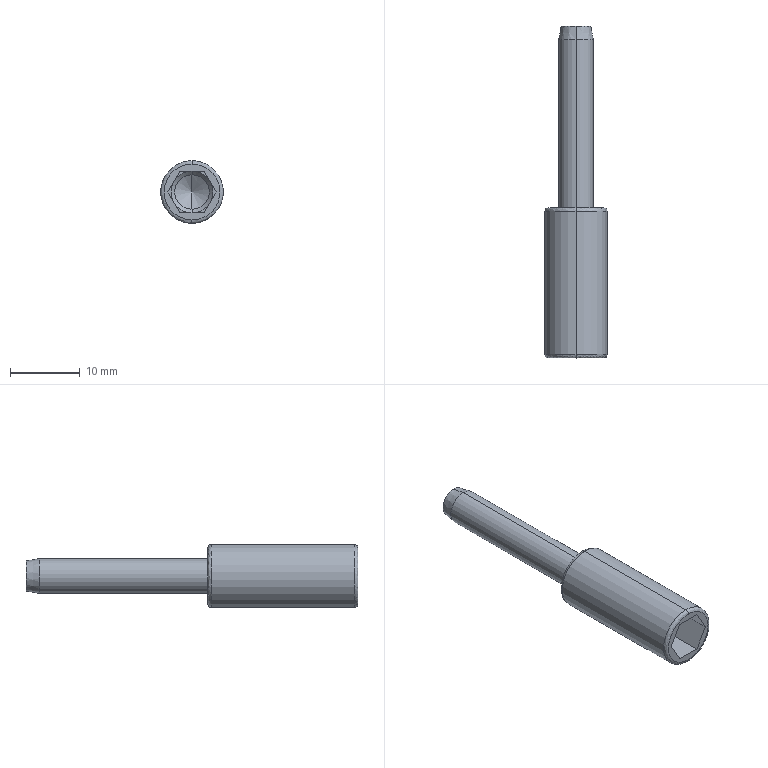Component | SolidWorks | HZ022-SE32x25S-1_HZ022-SE32x25S (10)-1 | 1 solid | 31 faces | box 9 x 47.5 x 9 mm | volume 1481 mm3 | plane 15 | cylinder 6 | cone 6 | spline 4 | commonest cylinder face diameters 9 x2 5 x2 4.917 x2 | material AL6061
STEP:
#1=COLOUR_RGB('',0.7922,0.8196,0.9333);
#2=FILL_AREA_STYLE_COLOUR('',#1);
#3=FILL_AREA_STYLE('',(#2));
#4=SURFACE_STYLE_FILL_AREA(#3);
#5=SURFACE_SIDE_STYLE('',(#4));
#6=SURFACE_STYLE_USAGE(.BOTH.,#5);
#7=PRESENTATION_STYLE_ASSIGNMENT((#6));
#8=CARTESIAN_POINT('',(-1.146,-5.555,13.976));
#9=VERTEX_POINT('',#8);
#10=CARTESIAN_POINT('',(-1.146,-5.555,13.661));
#11=VERTEX_POINT('',#10);
#12=CARTESIAN_POINT('',(-1.146,-5.555,13.976));
#13=CARTESIAN_POINT('',(-0.8313,-5.555,13.976));
#14=CARTESIAN_POINT('',(-0.8313,-5.555,13.661));
#15=CARTESIAN_POINT('',(-1.146,-5.555,13.661));
#16=(BOUNDED_CURVE()B_SPLINE_CURVE(3,(#12,#13,#14,#15),.UNSPECIFIED.,.F.,.F.)B_SPLINE_CURVE_WITH_KNOTS((4,4),(0.,1.),.UNSPECIFIED.)CURVE()GEOMETRIC_REPRESENTATION_ITEM()RATIONAL_B_SPLINE_CURVE((1.,0.3333,0.3333,1.))REPRESENTATION_ITEM(''));
#17=EDGE_CURVE('',#9,#11,#16,.T.);
#18=ORIENTED_EDGE('',*,*,#17,.T.);
#19=CARTESIAN_POINT('',(-1.146,-5.536,13.642));
#20=VERTEX_POINT('',#19);
#21=CARTESIAN_POINT('',(-1.146,-5.536,13.661));
#22=DIRECTION('',(1.,-0.,-0.));
#23=DIRECTION('',(0.,0.,-1.));
#24=AXIS2_PLACEMENT_3D('',#21,#22,#23);
#25=CIRCLE('',#24,0.01969);
#26=EDGE_CURVE('',#11,#20,#25,.T.);
#27=ORIENTED_EDGE('',*,*,#26,.T.);
#28=CARTESIAN_POINT('',(-1.146,-5.536,13.996));
#29=VERTEX_POINT('',#28);
#30=CARTESIAN_POINT('',(-1.146,-5.536,13.819));
#31=DIRECTION('',(0.,1.,0.));
#32=DIRECTION('',(0.,0.,1.));
#33=AXIS2_PLACEMENT_3D('',#30,#31,#32);
#34=CIRCLE('',#33,0.1772);
#35=EDGE_CURVE('',#29,#20,#34,.T.);
#36=ORIENTED_EDGE('',*,*,#35,.F.);
#37=CARTESIAN_POINT('',(-1.146,-5.536,13.976));
#38=DIRECTION('',(-1.,0.,0.));
#39=DIRECTION('',(0.,0.,1.));
#40=AXIS2_PLACEMENT_3D('',#37,#38,#39);
#41=CIRCLE('',#40,0.01969);
#42=EDGE_CURVE('',#9,#29,#41,.T.);
#43=ORIENTED_EDGE('',*,*,#42,.F.);
#44=EDGE_LOOP('',(#18,#27,#36,#43));
#45=FACE_OUTER_BOUND('',#44,.T.);
#46=CARTESIAN_POINT('',(-1.146,-5.555,13.661));
#47=CARTESIAN_POINT('',(-0.8313,-5.555,13.661));
#48=CARTESIAN_POINT('',(-0.8313,-5.555,13.976));
#49=CARTESIAN_POINT('',(-1.146,-5.555,13.976));
#50=CARTESIAN_POINT('',(-1.146,-5.555,13.65));
#51=CARTESIAN_POINT('',(-0.8082,-5.555,13.65));
#52=CARTESIAN_POINT('',(-0.8082,-5.555,13.988));
#53=CARTESIAN_POINT('',(-1.146,-5.555,13.988));
#54=CARTESIAN_POINT('',(-1.146,-5.547,13.642));
#55=CARTESIAN_POINT('',(-0.7919,-5.547,13.642));
#56=CARTESIAN_POINT('',(-0.7919,-5.547,13.996));
#57=CARTESIAN_POINT('',(-1.146,-5.547,13.996));
#58=CARTESIAN_POINT('',(-1.146,-5.536,13.642));
#59=CARTESIAN_POINT('',(-0.7919,-5.536,13.642));
#60=CARTESIAN_POINT('',(-0.7919,-5.536,13.996));
#61=CARTESIAN_POINT('',(-1.146,-5.536,13.996));
#62=(BOUNDED_SURFACE()B_SPLINE_SURFACE(3,3,((#46,#47,#48,#49),(#50,#51,#52,#53),(#54,#55,#56,#57),(#58,#59,#60,#61)),.UNSPECIFIED.,.F.,.F.,.T.)B_SPLINE_SURFACE_WITH_KNOTS((4,4),(4,4),(0.,1.),(0.,1.),.UNSPECIFIED.)GEOMETRIC_REPRESENTATION_ITEM()RATIONAL_B_SPLINE_SURFACE(((1.,0.3333,0.3333,1.),(0.8047,0.2682,0.2682,0.8047),(0.8047,0.2682,0.2682,0.8047),(1.,0.3333,0.3333,1.)))REPRESENTATION_ITEM('')SURFACE());
#63=ADVANCED_FACE('',(#45),#62,.T.);
#64=CARTESIAN_POINT('',(-1.146,-4.728,13.642));
#65=VERTEX_POINT('',#64);
#66=CARTESIAN_POINT('',(-1.146,-4.728,13.996));
#67=VERTEX_POINT('',#66);
#68=CARTESIAN_POINT('',(-1.146,-4.728,13.819));
#69=DIRECTION('',(-0.,-1.,-0.));
#70=DIRECTION('',(0.,0.,1.));
#71=AXIS2_PLACEMENT_3D('',#68,#69,#70);
#72=CIRCLE('',#71,0.1772);
#73=EDGE_CURVE('',#65,#67,#72,.T.);
#74=ORIENTED_EDGE('',*,*,#73,.F.);
#75=CARTESIAN_POINT('',(-1.146,-4.709,13.661));
#76=VERTEX_POINT('',#75);
#77=CARTESIAN_POINT('',(-1.146,-4.728,13.661));
#78=DIRECTION('',(1.,-0.,-0.));
#79=DIRECTION('',(0.,0.,-1.));
#80=AXIS2_PLACEMENT_3D('',#77,#78,#79);
#81=CIRCLE('',#80,0.01969);
#82=EDGE_CURVE('',#65,#76,#81,.T.);
#83=ORIENTED_EDGE('',*,*,#82,.T.);
#84=CARTESIAN_POINT('',(-1.146,-4.709,13.976));
#85=VERTEX_POINT('',#84);
#86=CARTESIAN_POINT('',(-1.146,-4.709,13.661));
#87=CARTESIAN_POINT('',(-0.8313,-4.709,13.661));
#88=CARTESIAN_POINT('',(-0.8313,-4.709,13.976));
#89=CARTESIAN_POINT('',(-1.146,-4.709,13.976));
#90=(BOUNDED_CURVE()B_SPLINE_CURVE(3,(#86,#87,#88,#89),.UNSPECIFIED.,.F.,.F.)B_SPLINE_CURVE_WITH_KNOTS((4,4),(0.,1.),.UNSPECIFIED.)CURVE()GEOMETRIC_REPRESENTATION_ITEM()RATIONAL_B_SPLINE_CURVE((1.,0.3333,0.3333,1.))REPRESENTATION_ITEM(''));
#91=EDGE_CURVE('',#76,#85,#90,.T.);
#92=ORIENTED_EDGE('',*,*,#91,.T.);
#93=CARTESIAN_POINT('',(-1.146,-4.728,13.976));
#94=DIRECTION('',(-1.,0.,0.));
#95=DIRECTION('',(0.,0.,1.));
#96=AXIS2_PLACEMENT_3D('',#93,#94,#95);
#97=CIRCLE('',#96,0.01969);
#98=EDGE_CURVE('',#67,#85,#97,.T.);
#99=ORIENTED_EDGE('',*,*,#98,.F.);
#100=EDGE_LOOP('',(#74,#83,#92,#99));
#101=FACE_OUTER_BOUND('',#100,.T.);
#102=CARTESIAN_POINT('',(-1.146,-4.728,13.642));
#103=CARTESIAN_POINT('',(-0.7919,-4.728,13.642));
#104=CARTESIAN_POINT('',(-0.7919,-4.728,13.996));
#105=CARTESIAN_POINT('',(-1.146,-4.728,13.996));
#106=CARTESIAN_POINT('',(-1.146,-4.717,13.642));
#107=CARTESIAN_POINT('',(-0.7919,-4.717,13.642));
#108=CARTESIAN_POINT('',(-0.7919,-4.717,13.996));
#109=CARTESIAN_POINT('',(-1.146,-4.717,13.996));
#110=CARTESIAN_POINT('',(-1.146,-4.709,13.65));
#111=CARTESIAN_POINT('',(-0.8082,-4.709,13.65));
#112=CARTESIAN_POINT('',(-0.8082,-4.709,13.988));
#113=CARTESIAN_POINT('',(-1.146,-4.709,13.988));
#114=CARTESIAN_POINT('',(-1.146,-4.709,13.661));
#115=CARTESIAN_POINT('',(-0.8313,-4.709,13.661));
#116=CARTESIAN_POINT('',(-0.8313,-4.709,13.976));
#117=CARTESIAN_POINT('',(-1.146,-4.709,13.976));
#118=(BOUNDED_SURFACE()B_SPLINE_SURFACE(3,3,((#102,#103,#104,#105),(#106,#107,#108,#109),(#110,#111,#112,#113),(#114,#115,#116,#117)),.UNSPECIFIED.,.F.,.F.,.F.)B_SPLINE_SURFACE_WITH_KNOTS((4,4),(4,4),(0.,1.),(0.,1.),.UNSPECIFIED.)GEOMETRIC_REPRESENTATION_ITEM()RATIONAL_B_SPLINE_SURFACE(((1.,0.3333,0.3333,1.),(0.8047,0.2682,0.2682,0.8047),(0.8047,0.2682,0.2682,0.8047),(1.,0.3333,0.3333,1.)))REPRESENTATION_ITEM('')SURFACE());
#119=ADVANCED_FACE('',(#101),#118,.T.);
#120=ORIENTED_EDGE('',*,*,#35,.T.);
#121=CARTESIAN_POINT('',(-1.146,-5.132,13.642));
#122=DIRECTION('',(0.,1.,0.));
#123=VECTOR('',#122,39.37);
#124=LINE('',#121,#123);
#125=EDGE_CURVE('',#20,#65,#124,.T.);
#126=ORIENTED_EDGE('',*,*,#125,.T.);
#127=ORIENTED_EDGE('',*,*,#73,.T.);
#128=CARTESIAN_POINT('',(-1.146,-5.132,13.996));
#129=DIRECTION('',(0.,1.,0.));
#130=VECTOR('',#129,39.37);
#131=LINE('',#128,#130);
#132=EDGE_CURVE('',#29,#67,#131,.T.);
#133=ORIENTED_EDGE('',*,*,#132,.F.);
#134=EDGE_LOOP('',(#120,#126,#127,#133));
#135=FACE_OUTER_BOUND('',#134,.T.);
#136=CARTESIAN_POINT('',(-1.146,-5.132,13.819));
#137=DIRECTION('',(0.,1.,0.));
#138=DIRECTION('',(0.,0.,1.));
#139=AXIS2_PLACEMENT_3D('',#136,#137,#138);
#140=CYLINDRICAL_SURFACE('',#139,0.1772);
#141=ADVANCED_FACE('',(#135),#140,.T.);
#142=CARTESIAN_POINT('',(-1.146,-4.709,13.72));
#143=VERTEX_POINT('',#142);
#144=CARTESIAN_POINT('',(-1.146,-4.709,13.917));
#145=VERTEX_POINT('',#144);
#146=CARTESIAN_POINT('',(-1.146,-4.709,13.819));
#147=DIRECTION('',(-0.,-1.,-0.));
#148=DIRECTION('',(0.,0.,1.));
#149=AXIS2_PLACEMENT_3D('',#146,#147,#148);
#150=CIRCLE('',#149,0.09843);
#151=EDGE_CURVE('',#143,#145,#150,.T.);
#152=ORIENTED_EDGE('',*,*,#151,.F.);
#153=CARTESIAN_POINT('',(-1.146,-3.762,13.72));
#154=VERTEX_POINT('',#153);
#155=CARTESIAN_POINT('',(-1.146,-4.235,13.72));
#156=DIRECTION('',(0.,1.,0.));
#157=VECTOR('',#156,39.37);
#158=LINE('',#155,#157);
#159=EDGE_CURVE('',#143,#154,#158,.T.);
#160=ORIENTED_EDGE('',*,*,#159,.T.);
#161=CARTESIAN_POINT('',(-1.146,-3.762,13.917));
#162=VERTEX_POINT('',#161);
#163=CARTESIAN_POINT('',(-1.146,-3.762,13.819));
#164=DIRECTION('',(-0.,-1.,-0.));
#165=DIRECTION('',(0.,0.,1.));
#166=AXIS2_PLACEMENT_3D('',#163,#164,#165);
#167=CIRCLE('',#166,0.09843);
#168=EDGE_CURVE('',#154,#162,#167,.T.);
#169=ORIENTED_EDGE('',*,*,#168,.T.);
#170=CARTESIAN_POINT('',(-1.146,-4.235,13.917));
#171=DIRECTION('',(0.,1.,0.));
#172=VECTOR('',#171,39.37);
#173=LINE('',#170,#172);
#174=EDGE_CURVE('',#145,#162,#173,.T.);
#175=ORIENTED_EDGE('',*,*,#174,.F.);
#176=EDGE_LOOP('',(#152,#160,#169,#175));
#177=FACE_OUTER_BOUND('',#176,.T.);
#178=CARTESIAN_POINT('',(-1.146,-4.235,13.819));
#179=DIRECTION('',(0.,1.,0.));
#180=DIRECTION('',(0.,0.,1.));
#181=AXIS2_PLACEMENT_3D('',#178,#179,#180);
#182=CYLINDRICAL_SURFACE('',#181,0.09843);
#183=ADVANCED_FACE('',(#177),#182,.T.);
#184=CARTESIAN_POINT('',(-1.146,-3.685,13.734));
#185=VERTEX_POINT('',#184);
#186=CARTESIAN_POINT('',(-1.146,-3.685,13.904));
#187=VERTEX_POINT('',#186);
#188=CARTESIAN_POINT('',(-1.146,-3.685,13.819));
#189=DIRECTION('',(-0.,-1.,-0.));
#190=DIRECTION('',(0.,0.,-1.));
#191=AXIS2_PLACEMENT_3D('',#188,#189,#190);
#192=CIRCLE('',#191,0.08484);
#193=EDGE_CURVE('',#185,#187,#192,.T.);
#194=ORIENTED_EDGE('',*,*,#193,.T.);
#195=CARTESIAN_POINT('',(-1.146,-3.762,13.917));
#196=DIRECTION('',(-0.,-0.9848,0.1736));
#197=VECTOR('',#196,39.37);
#198=LINE('',#195,#197);
#199=EDGE_CURVE('',#187,#162,#198,.T.);
#200=ORIENTED_EDGE('',*,*,#199,.T.);
#201=ORIENTED_EDGE('',*,*,#168,.F.);
#202=CARTESIAN_POINT('',(-1.146,-3.762,13.72));
#203=DIRECTION('',(-0.,-0.9848,-0.1736));
#204=VECTOR('',#203,39.37);
#205=LINE('',#202,#204);
#206=EDGE_CURVE('',#185,#154,#205,.T.);
#207=ORIENTED_EDGE('',*,*,#206,.F.);
#208=EDGE_LOOP('',(#194,#200,#201,#207));
#209=FACE_OUTER_BOUND('',#208,.T.);
#210=CARTESIAN_POINT('',(-1.146,-3.762,13.819));
#211=DIRECTION('',(-0.,-1.,-0.));
#212=DIRECTION('',(0.,0.,-1.));
#213=AXIS2_PLACEMENT_3D('',#210,#211,#212);
#214=CONICAL_SURFACE('',#213,0.09843,0.1745);
#215=ADVANCED_FACE('',(#209),#214,.T.);
#216=CARTESIAN_POINT('',(-1.146,-5.357,13.916));
#217=VERTEX_POINT('',#216);
#218=CARTESIAN_POINT('',(-1.146,-5.357,13.722));
#219=VERTEX_POINT('',#218);
#220=CARTESIAN_POINT('',(-1.146,-5.357,13.819));
#221=DIRECTION('',(-0.,-1.,-0.));
#222=DIRECTION('',(-1.,0.,0.));
#223=AXIS2_PLACEMENT_3D('',#220,#221,#222);
#224=CIRCLE('',#223,0.09679);
#225=EDGE_CURVE('',#217,#219,#224,.T.);
#226=ORIENTED_EDGE('',*,*,#225,.F.);
#227=CARTESIAN_POINT('',(-1.146,-5.378,13.937));
#228=VERTEX_POINT('',#227);
#229=CARTESIAN_POINT('',(-1.146,-5.378,13.937));
#230=DIRECTION('',(-0.,-0.7071,0.7071));
#231=VECTOR('',#230,39.37);
#232=LINE('',#229,#231);
#233=EDGE_CURVE('',#217,#228,#232,.T.);
#234=ORIENTED_EDGE('',*,*,#233,.T.);
#235=CARTESIAN_POINT('',(-1.249,-5.378,13.878));
#236=VERTEX_POINT('',#235);
#237=CARTESIAN_POINT('',(-1.146,-5.378,13.819));
#238=DIRECTION('',(-0.,-1.,-0.));
#239=DIRECTION('',(0.,0.,-1.));
#240=AXIS2_PLACEMENT_3D('',#237,#238,#239);
#241=CIRCLE('',#240,0.1181);
#242=EDGE_CURVE('',#228,#236,#241,.T.);
#243=ORIENTED_EDGE('',*,*,#242,.T.);
#244=CARTESIAN_POINT('',(-1.249,-5.378,13.76));
#245=VERTEX_POINT('',#244);
#246=CARTESIAN_POINT('',(-1.146,-5.378,13.819));
#247=DIRECTION('',(0.,1.,0.));
#248=DIRECTION('',(-0.,0.,-1.));
#249=AXIS2_PLACEMENT_3D('',#246,#247,#248);
#250=CIRCLE('',#249,0.1181);
#251=EDGE_CURVE('',#245,#236,#250,.T.);
#252=ORIENTED_EDGE('',*,*,#251,.F.);
#253=CARTESIAN_POINT('',(-1.146,-5.378,13.701));
#254=VERTEX_POINT('',#253);
#255=CARTESIAN_POINT('',(-1.146,-5.378,13.819));
#256=DIRECTION('',(0.,1.,0.));
#257=DIRECTION('',(0.,0.,-1.));
#258=AXIS2_PLACEMENT_3D('',#255,#256,#257);
#259=CIRCLE('',#258,0.1181);
#260=EDGE_CURVE('',#254,#245,#259,.T.);
#261=ORIENTED_EDGE('',*,*,#260,.F.);
#262=CARTESIAN_POINT('',(-1.146,-5.378,13.701));
#263=DIRECTION('',(-0.,-0.7071,-0.7071));
#264=VECTOR('',#263,39.37);
#265=LINE('',#262,#264);
#266=EDGE_CURVE('',#219,#254,#265,.T.);
#267=ORIENTED_EDGE('',*,*,#266,.F.);
#268=EDGE_LOOP('',(#226,#234,#243,#252,#261,#267));
#269=FACE_OUTER_BOUND('',#268,.T.);
#270=CARTESIAN_POINT('',(-1.146,-5.378,13.819));
#271=DIRECTION('',(-0.,-1.,-0.));
#272=DIRECTION('',(0.,0.,-1.));
#273=AXIS2_PLACEMENT_3D('',#270,#271,#272);
#274=CONICAL_SURFACE('',#273,0.1181,0.7854);
#275=ADVANCED_FACE('',(#269),#274,.F.);
#276=ORIENTED_EDGE('',*,*,#225,.T.);
#277=CARTESIAN_POINT('',(-1.146,-4.886,13.722));
#278=VERTEX_POINT('',#277);
#279=CARTESIAN_POINT('',(-1.146,-5.121,13.722));
#280=DIRECTION('',(0.,1.,0.));
#281=VECTOR('',#280,39.37);
#282=LINE('',#279,#281);
#283=EDGE_CURVE('',#219,#278,#282,.T.);
#284=ORIENTED_EDGE('',*,*,#283,.T.);
#285=CARTESIAN_POINT('',(-1.146,-4.886,13.916));
#286=VERTEX_POINT('',#285);
#287=CARTESIAN_POINT('',(-1.146,-4.886,13.819));
#288=DIRECTION('',(-0.,-1.,-0.));
#289=DIRECTION('',(0.,0.,1.));
#290=AXIS2_PLACEMENT_3D('',#287,#288,#289);
#291=CIRCLE('',#290,0.09679);
#292=EDGE_CURVE('',#286,#278,#291,.T.);
#293=ORIENTED_EDGE('',*,*,#292,.F.);
#294=CARTESIAN_POINT('',(-1.146,-5.121,13.916));
#295=DIRECTION('',(0.,1.,0.));
#296=VECTOR('',#295,39.37);
#297=LINE('',#294,#296);
#298=EDGE_CURVE('',#217,#286,#297,.T.);
#299=ORIENTED_EDGE('',*,*,#298,.F.);
#300=EDGE_LOOP('',(#276,#284,#293,#299));
#301=FACE_OUTER_BOUND('',#300,.T.);
#302=CARTESIAN_POINT('',(-1.146,-5.121,13.819));
#303=DIRECTION('',(0.,1.,0.));
#304=DIRECTION('',(0.,0.,1.));
#305=AXIS2_PLACEMENT_3D('',#302,#303,#304);
#306=CYLINDRICAL_SURFACE('',#305,0.09679);
#307=ADVANCED_FACE('',(#301),#306,.F.);
#308=CARTESIAN_POINT('',(-1.146,-4.83,13.819));
#309=VERTEX_POINT('',#308);
#310=CARTESIAN_POINT('',(-1.146,-4.886,13.722));
#311=DIRECTION('',(-0.,-0.5,-0.866));
#312=VECTOR('',#311,39.37);
#313=LINE('',#310,#312);
#314=EDGE_CURVE('',#309,#278,#313,.T.);
#315=ORIENTED_EDGE('',*,*,#314,.F.);
#316=CARTESIAN_POINT('',(-1.146,-4.886,13.916));
#317=DIRECTION('',(-0.,-0.5,0.866));
#318=VECTOR('',#317,39.37);
#319=LINE('',#316,#318);
#320=EDGE_CURVE('',#309,#286,#319,.T.);
#321=ORIENTED_EDGE('',*,*,#320,.T.);
#322=ORIENTED_EDGE('',*,*,#292,.T.);
#323=EDGE_LOOP('',(#315,#321,#322));
#324=FACE_OUTER_BOUND('',#323,.T.);
#325=CARTESIAN_POINT('',(-1.146,-4.886,13.819));
#326=DIRECTION('',(-0.,-1.,-0.));
#327=DIRECTION('',(0.,0.,-1.));
#328=AXIS2_PLACEMENT_3D('',#325,#326,#327);
#329=CONICAL_SURFACE('',#328,0.09679,1.047);
#330=ADVANCED_FACE('',(#324),#329,.F.);
#331=ORIENTED_EDGE('',*,*,#125,.F.);
#332=CARTESIAN_POINT('',(-1.146,-5.536,13.819));
#333=DIRECTION('',(0.,1.,0.));
#334=DIRECTION('',(0.,0.,1.));
#335=AXIS2_PLACEMENT_3D('',#332,#333,#334);
#336=CIRCLE('',#335,0.1772);
#337=EDGE_CURVE('',#20,#29,#336,.T.);
#338=ORIENTED_EDGE('',*,*,#337,.T.);
#339=ORIENTED_EDGE('',*,*,#132,.T.);
#340=CARTESIAN_POINT('',(-1.146,-4.728,13.819));
#341=DIRECTION('',(-0.,-1.,-0.));
#342=DIRECTION('',(0.,0.,1.));
#343=AXIS2_PLACEMENT_3D('',#340,#341,#342);
#344=CIRCLE('',#343,0.1772);
#345=EDGE_CURVE('',#67,#65,#344,.T.);
#346=ORIENTED_EDGE('',*,*,#345,.T.);
#347=EDGE_LOOP('',(#331,#338,#339,#346));
#348=FACE_OUTER_BOUND('',#347,.T.);
#349=CARTESIAN_POINT('',(-1.146,-5.132,13.819));
#350=DIRECTION('',(0.,1.,0.));
#351=DIRECTION('',(0.,0.,1.));
#352=AXIS2_PLACEMENT_3D('',#349,#350,#351);
#353=CYLINDRICAL_SURFACE('',#352,0.1772);
#354=ADVANCED_FACE('',(#348),#353,.T.);
#355=ORIENTED_EDGE('',*,*,#26,.F.);
#356=CARTESIAN_POINT('',(-1.304,-5.555,13.819));
#357=VERTEX_POINT('',#356);
#358=CARTESIAN_POINT('',(-1.146,-5.555,13.661));
#359=CARTESIAN_POINT('',(-1.239,-5.555,13.661));
#360=CARTESIAN_POINT('',(-1.304,-5.555,13.727));
#361=CARTESIAN_POINT('',(-1.304,-5.555,13.819));
#362=(BOUNDED_CURVE()B_SPLINE_CURVE(3,(#358,#359,#360,#361),.UNSPECIFIED.,.F.,.F.)B_SPLINE_CURVE_WITH_KNOTS((4,4),(0.,1.),.UNSPECIFIED.)CURVE()GEOMETRIC_REPRESENTATION_ITEM()RATIONAL_B_SPLINE_CURVE((1.,0.8047,0.8047,1.))REPRESENTATION_ITEM(''));
#363=EDGE_CURVE('',#11,#357,#362,.T.);
#364=ORIENTED_EDGE('',*,*,#363,.T.);
#365=CARTESIAN_POINT('',(-1.304,-5.555,13.819));
#366=CARTESIAN_POINT('',(-1.304,-5.555,13.911));
#367=CARTESIAN_POINT('',(-1.239,-5.555,13.976));
#368=CARTESIAN_POINT('',(-1.146,-5.555,13.976));
#369=(BOUNDED_CURVE()B_SPLINE_CURVE(3,(#365,#366,#367,#368),.UNSPECIFIED.,.F.,.F.)B_SPLINE_CURVE_WITH_KNOTS((4,4),(0.,1.),.UNSPECIFIED.)CURVE()GEOMETRIC_REPRESENTATION_ITEM()RATIONAL_B_SPLINE_CURVE((1.,0.8047,0.8047,1.))REPRESENTATION_ITEM(''));
#370=EDGE_CURVE('',#357,#9,#369,.T.);
#371=ORIENTED_EDGE('',*,*,#370,.T.);
#372=ORIENTED_EDGE('',*,*,#42,.T.);
#373=ORIENTED_EDGE('',*,*,#337,.F.);
#374=EDGE_LOOP('',(#355,#364,#371,#372,#373));
#375=FACE_OUTER_BOUND('',#374,.T.);
#376=CARTESIAN_POINT('',(-1.146,-5.555,13.976));
#377=CARTESIAN_POINT('',(-1.461,-5.555,13.976));
#378=CARTESIAN_POINT('',(-1.461,-5.555,13.661));
#379=CARTESIAN_POINT('',(-1.146,-5.555,13.661));
#380=CARTESIAN_POINT('',(-1.146,-5.555,13.988));
#381=CARTESIAN_POINT('',(-1.484,-5.555,13.988));
#382=CARTESIAN_POINT('',(-1.484,-5.555,13.65));
#383=CARTESIAN_POINT('',(-1.146,-5.555,13.65));
#384=CARTESIAN_POINT('',(-1.146,-5.547,13.996));
#385=CARTESIAN_POINT('',(-1.501,-5.547,13.996));
#386=CARTESIAN_POINT('',(-1.501,-5.547,13.642));
#387=CARTESIAN_POINT('',(-1.146,-5.547,13.642));
#388=CARTESIAN_POINT('',(-1.146,-5.536,13.996));
#389=CARTESIAN_POINT('',(-1.501,-5.536,13.996));
#390=CARTESIAN_POINT('',(-1.501,-5.536,13.642));
#391=CARTESIAN_POINT('',(-1.146,-5.536,13.642));
#392=(BOUNDED_SURFACE()B_SPLINE_SURFACE(3,3,((#376,#377,#378,#379),(#380,#381,#382,#383),(#384,#385,#386,#387),(#388,#389,#390,#391)),.UNSPECIFIED.,.F.,.F.,.F.)B_SPLINE_SURFACE_WITH_KNOTS((4,4),(4,4),(0.,1.),(0.,1.),.UNSPECIFIED.)GEOMETRIC_REPRESENTATION_ITEM()RATIONAL_B_SPLINE_SURFACE(((1.,0.3333,0.3333,1.),(0.8047,0.2682,0.2682,0.8047),(0.8047,0.2682,0.2682,0.8047),(1.,0.3333,0.3333,1.)))REPRESENTATION_ITEM('')SURFACE());
#393=ADVANCED_FACE('',(#375),#392,.T.);
#394=ORIENTED_EDGE('',*,*,#82,.F.);
#395=ORIENTED_EDGE('',*,*,#345,.F.);
#396=ORIENTED_EDGE('',*,*,#98,.T.);
#397=CARTESIAN_POINT('',(-1.304,-4.709,13.819));
#398=VERTEX_POINT('',#397);
#399=CARTESIAN_POINT('',(-1.146,-4.709,13.976));
#400=CARTESIAN_POINT('',(-1.239,-4.709,13.976));
#401=CARTESIAN_POINT('',(-1.304,-4.709,13.911));
#402=CARTESIAN_POINT('',(-1.304,-4.709,13.819));
#403=(BOUNDED_CURVE()B_SPLINE_CURVE(3,(#399,#400,#401,#402),.UNSPECIFIED.,.F.,.F.)B_SPLINE_CURVE_WITH_KNOTS((4,4),(0.,1.),.UNSPECIFIED.)CURVE()GEOMETRIC_REPRESENTATION_ITEM()RATIONAL_B_SPLINE_CURVE((1.,0.8047,0.8047,1.))REPRESENTATION_ITEM(''));
#404=EDGE_CURVE('',#85,#398,#403,.T.);
#405=ORIENTED_EDGE('',*,*,#404,.T.);
#406=CARTESIAN_POINT('',(-1.304,-4.709,13.819));
#407=CARTESIAN_POINT('',(-1.304,-4.709,13.727));
#408=CARTESIAN_POINT('',(-1.239,-4.709,13.661));
#409=CARTESIAN_POINT('',(-1.146,-4.709,13.661));
#410=(BOUNDED_CURVE()B_SPLINE_CURVE(3,(#406,#407,#408,#409),.UNSPECIFIED.,.F.,.F.)B_SPLINE_CURVE_WITH_KNOTS((4,4),(0.,1.),.UNSPECIFIED.)CURVE()GEOMETRIC_REPRESENTATION_ITEM()RATIONAL_B_SPLINE_CURVE((1.,0.8047,0.8047,1.))REPRESENTATION_ITEM(''));
#411=EDGE_CURVE('',#398,#76,#410,.T.);
#412=ORIENTED_EDGE('',*,*,#411,.T.);
#413=EDGE_LOOP('',(#394,#395,#396,#405,#412));
#414=FACE_OUTER_BOUND('',#413,.T.);
#415=CARTESIAN_POINT('',(-1.146,-4.728,13.996));
#416=CARTESIAN_POINT('',(-1.501,-4.728,13.996));
#417=CARTESIAN_POINT('',(-1.501,-4.728,13.642));
#418=CARTESIAN_POINT('',(-1.146,-4.728,13.642));
#419=CARTESIAN_POINT('',(-1.146,-4.717,13.996));
#420=CARTESIAN_POINT('',(-1.501,-4.717,13.996));
#421=CARTESIAN_POINT('',(-1.501,-4.717,13.642));
#422=CARTESIAN_POINT('',(-1.146,-4.717,13.642));
#423=CARTESIAN_POINT('',(-1.146,-4.709,13.988));
#424=CARTESIAN_POINT('',(-1.484,-4.709,13.988));
#425=CARTESIAN_POINT('',(-1.484,-4.709,13.65));
#426=CARTESIAN_POINT('',(-1.146,-4.709,13.65));
#427=CARTESIAN_POINT('',(-1.146,-4.709,13.976));
#428=CARTESIAN_POINT('',(-1.461,-4.709,13.976));
#429=CARTESIAN_POINT('',(-1.461,-4.709,13.661));
#430=CARTESIAN_POINT('',(-1.146,-4.709,13.661));
#431=(BOUNDED_SURFACE()B_SPLINE_SURFACE(3,3,((#415,#416,#417,#418),(#419,#420,#421,#422),(#423,#424,#425,#426),(#427,#428,#429,#430)),.UNSPECIFIED.,.F.,.F.,.F.)B_SPLINE_SURFACE_WITH_KNOTS((4,4),(4,4),(0.,1.),(0.,1.),.UNSPECIFIED.)GEOMETRIC_REPRESENTATION_ITEM()RATIONAL_B_SPLINE_SURFACE(((1.,0.3333,0.3333,1.),(0.8047,0.2682,0.2682,0.8047),(0.8047,0.2682,0.2682,0.8047),(1.,0.3333,0.3333,1.)))REPRESENTATION_ITEM('')SURFACE());
#432=ADVANCED_FACE('',(#414),#431,.T.);
#433=ORIENTED_EDGE('',*,*,#17,.F.);
#434=ORIENTED_EDGE('',*,*,#370,.F.);
#435=ORIENTED_EDGE('',*,*,#363,.F.);
#436=EDGE_LOOP('',(#433,#434,#435));
#437=FACE_OUTER_BOUND('',#436,.T.);
#438=CARTESIAN_POINT('',(-1.078,-5.555,13.701));
#439=VERTEX_POINT('',#438);
#440=CARTESIAN_POINT('',(-1.214,-5.555,13.701));
#441=VERTEX_POINT('',#440);
#442=CARTESIAN_POINT('',(-1.225,-5.555,13.701));
#443=DIRECTION('',(-1.,0.,0.));
#444=VECTOR('',#443,39.37);
#445=LINE('',#442,#444);
#446=EDGE_CURVE('',#439,#441,#445,.T.);
#447=ORIENTED_EDGE('',*,*,#446,.T.);
#448=CARTESIAN_POINT('',(-1.283,-5.555,13.819));
#449=VERTEX_POINT('',#448);
#450=CARTESIAN_POINT('',(-1.214,-5.555,13.701));
#451=DIRECTION('',(-0.5,0.,0.866));
#452=VECTOR('',#451,39.37);
#453=LINE('',#450,#452);
#454=EDGE_CURVE('',#441,#449,#453,.T.);
#455=ORIENTED_EDGE('',*,*,#454,.T.);
#456=CARTESIAN_POINT('',(-1.214,-5.555,13.937));
#457=VERTEX_POINT('',#456);
#458=CARTESIAN_POINT('',(-1.283,-5.555,13.819));
#459=DIRECTION('',(0.5,-0.,0.866));
#460=VECTOR('',#459,39.37);
#461=LINE('',#458,#460);
#462=EDGE_CURVE('',#449,#457,#461,.T.);
#463=ORIENTED_EDGE('',*,*,#462,.T.);
#464=CARTESIAN_POINT('',(-1.078,-5.555,13.937));
#465=VERTEX_POINT('',#464);
#466=CARTESIAN_POINT('',(-1.225,-5.555,13.937));
#467=DIRECTION('',(1.,-0.,-0.));
#468=VECTOR('',#467,39.37);
#469=LINE('',#466,#468);
#470=EDGE_CURVE('',#457,#465,#469,.T.);
#471=ORIENTED_EDGE('',*,*,#470,.T.);
#472=CARTESIAN_POINT('',(-1.01,-5.555,13.819));
#473=VERTEX_POINT('',#472);
#474=CARTESIAN_POINT('',(-1.078,-5.555,13.937));
#475=DIRECTION('',(0.5,-0.,-0.866));
#476=VECTOR('',#475,39.37);
#477=LINE('',#474,#476);
#478=EDGE_CURVE('',#465,#473,#477,.T.);
#479=ORIENTED_EDGE('',*,*,#478,.T.);
#480=CARTESIAN_POINT('',(-1.01,-5.555,13.819));
#481=DIRECTION('',(-0.5,0.,-0.866));
#482=VECTOR('',#481,39.37);
#483=LINE('',#480,#482);
#484=EDGE_CURVE('',#473,#439,#483,.T.);
#485=ORIENTED_EDGE('',*,*,#484,.T.);
#486=EDGE_LOOP('',(#447,#455,#463,#471,#479,#485));
#487=FACE_BOUND('',#486,.T.);
#488=CARTESIAN_POINT('',(-1.225,-5.555,13.819));
#489=DIRECTION('',(-0.,-1.,-0.));
#490=DIRECTION('',(-0.,0.,-1.));
#491=AXIS2_PLACEMENT_3D('',#488,#489,#490);
#492=PLANE('',#491);
#493=ADVANCED_FACE('',(#437,#487),#492,.T.);
#494=CARTESIAN_POINT('',(-1.146,-4.709,13.819));
#495=DIRECTION('',(-0.,-1.,-0.));
#496=DIRECTION('',(0.,0.,1.));
#497=AXIS2_PLACEMENT_3D('',#494,#495,#496);
#498=CIRCLE('',#497,0.09843);
#499=EDGE_CURVE('',#145,#143,#498,.T.);
#500=ORIENTED_EDGE('',*,*,#499,.T.);
#501=ORIENTED_EDGE('',*,*,#151,.T.);
#502=EDGE_LOOP('',(#500,#501));
#503=FACE_BOUND('',#502,.T.);
#504=ORIENTED_EDGE('',*,*,#404,.F.);
#505=ORIENTED_EDGE('',*,*,#91,.F.);
#506=ORIENTED_EDGE('',*,*,#411,.F.);
#507=EDGE_LOOP('',(#504,#505,#506));
#508=FACE_OUTER_BOUND('',#507,.T.);
#509=CARTESIAN_POINT('',(-1.225,-4.709,13.819));
#510=DIRECTION('',(0.,1.,0.));
#511=DIRECTION('',(-1.,0.,0.));
#512=AXIS2_PLACEMENT_3D('',#509,#510,#511);
#513=PLANE('',#512);
#514=ADVANCED_FACE('',(#503,#508),#513,.T.);
#515=CARTESIAN_POINT('',(-1.283,-5.378,13.819));
#516=VERTEX_POINT('',#515);
#517=CARTESIAN_POINT('',(-1.283,-5.555,13.819));
#518=DIRECTION('',(0.,1.,0.));
#519=VECTOR('',#518,39.37);
#520=LINE('',#517,#519);
#521=EDGE_CURVE('',#449,#516,#520,.T.);
#522=ORIENTED_EDGE('',*,*,#521,.F.);
#523=ORIENTED_EDGE('',*,*,#454,.F.);
#524=CARTESIAN_POINT('',(-1.214,-5.378,13.701));
#525=VERTEX_POINT('',#524);
#526=CARTESIAN_POINT('',(-1.214,-5.555,13.701));
#527=DIRECTION('',(-0.,-1.,-0.));
#528=VECTOR('',#527,39.37);
#529=LINE('',#526,#528);
#530=EDGE_CURVE('',#525,#441,#529,.T.);
#531=ORIENTED_EDGE('',*,*,#530,.F.);
#532=CARTESIAN_POINT('',(-1.214,-5.378,13.701));
#533=DIRECTION('',(-0.5,0.,0.866));
#534=VECTOR('',#533,39.37);
#535=LINE('',#532,#534);
#536=EDGE_CURVE('',#525,#245,#535,.T.);
#537=ORIENTED_EDGE('',*,*,#536,.T.);
#538=CARTESIAN_POINT('',(-1.283,-5.378,13.819));
#539=DIRECTION('',(0.5,-0.,-0.866));
#540=VECTOR('',#539,39.37);
#541=LINE('',#538,#540);
#542=EDGE_CURVE('',#516,#245,#541,.T.);
#543=ORIENTED_EDGE('',*,*,#542,.F.);
#544=EDGE_LOOP('',(#522,#523,#531,#537,#543));
#545=FACE_OUTER_BOUND('',#544,.T.);
#546=CARTESIAN_POINT('',(-1.283,-5.555,13.819));
#547=DIRECTION('',(-0.866,0.,-0.5));
#548=DIRECTION('',(0.5,-0.,-0.866));
#549=AXIS2_PLACEMENT_3D('',#546,#547,#548);
#550=PLANE('',#549);
#551=ADVANCED_FACE('',(#545),#550,.F.);
#552=ORIENTED_EDGE('',*,*,#530,.T.);
#553=ORIENTED_EDGE('',*,*,#446,.F.);
#554=CARTESIAN_POINT('',(-1.078,-5.378,13.701));
#555=VERTEX_POINT('',#554);
#556=CARTESIAN_POINT('',(-1.078,-5.555,13.701));
#557=DIRECTION('',(-0.,-1.,-0.));
#558=VECTOR('',#557,39.37);
#559=LINE('',#556,#558);
#560=EDGE_CURVE('',#555,#439,#559,.T.);
#561=ORIENTED_EDGE('',*,*,#560,.F.);
#562=CARTESIAN_POINT('',(-1.146,-5.378,13.701));
#563=DIRECTION('',(-1.,0.,0.));
#564=VECTOR('',#563,39.37);
#565=LINE('',#562,#564);
#566=EDGE_CURVE('',#555,#254,#565,.T.);
#567=ORIENTED_EDGE('',*,*,#566,.T.);
#568=CARTESIAN_POINT('',(-1.146,-5.378,13.701));
#569=DIRECTION('',(-1.,0.,0.));
#570=VECTOR('',#569,39.37);
#571=LINE('',#568,#570);
#572=EDGE_CURVE('',#254,#525,#571,.T.);
#573=ORIENTED_EDGE('',*,*,#572,.T.);
#574=EDGE_LOOP('',(#552,#553,#561,#567,#573));
#575=FACE_OUTER_BOUND('',#574,.T.);
#576=CARTESIAN_POINT('',(-1.214,-5.555,13.701));
#577=DIRECTION('',(-0.,0.,-1.));
#578=DIRECTION('',(0.,1.,0.));
#579=AXIS2_PLACEMENT_3D('',#576,#577,#578);
#580=PLANE('',#579);
#581=ADVANCED_FACE('',(#575),#580,.F.);
#582=ORIENTED_EDGE('',*,*,#560,.T.);
#583=ORIENTED_EDGE('',*,*,#484,.F.);
#584=CARTESIAN_POINT('',(-1.01,-5.378,13.819));
#585=VERTEX_POINT('',#584);
#586=CARTESIAN_POINT('',(-1.01,-5.555,13.819));
#587=DIRECTION('',(-0.,-1.,-0.));
#588=VECTOR('',#587,39.37);
#589=LINE('',#586,#588);
#590=EDGE_CURVE('',#585,#473,#589,.T.);
#591=ORIENTED_EDGE('',*,*,#590,.F.);
#592=CARTESIAN_POINT('',(-1.044,-5.378,13.76));
#593=VERTEX_POINT('',#592);
#594=CARTESIAN_POINT('',(-1.078,-5.378,13.701));
#595=DIRECTION('',(0.5,-0.,0.866));
#596=VECTOR('',#595,39.37);
#597=LINE('',#594,#596);
#598=EDGE_CURVE('',#593,#585,#597,.T.);
#599=ORIENTED_EDGE('',*,*,#598,.F.);
#600=CARTESIAN_POINT('',(-1.044,-5.378,13.76));
#601=DIRECTION('',(-0.5,0.,-0.866));
#602=VECTOR('',#601,39.37);
#603=LINE('',#600,#602);
#604=EDGE_CURVE('',#593,#555,#603,.T.);
#605=ORIENTED_EDGE('',*,*,#604,.T.);
#606=EDGE_LOOP('',(#582,#583,#591,#599,#605));
#607=FACE_OUTER_BOUND('',#606,.T.);
#608=CARTESIAN_POINT('',(-1.078,-5.555,13.701));
#609=DIRECTION('',(0.866,-0.,-0.5));
#610=DIRECTION('',(0.5,-0.,0.866));
#611=AXIS2_PLACEMENT_3D('',#608,#609,#610);
#612=PLANE('',#611);
#613=ADVANCED_FACE('',(#607),#612,.F.);
#614=ORIENTED_EDGE('',*,*,#590,.T.);
#615=ORIENTED_EDGE('',*,*,#478,.F.);
#616=CARTESIAN_POINT('',(-1.078,-5.378,13.937));
#617=VERTEX_POINT('',#616);
#618=CARTESIAN_POINT('',(-1.078,-5.555,13.937));
#619=DIRECTION('',(-0.,-1.,-0.));
#620=VECTOR('',#619,39.37);
#621=LINE('',#618,#620);
#622=EDGE_CURVE('',#617,#465,#621,.T.);
#623=ORIENTED_EDGE('',*,*,#622,.F.);
#624=CARTESIAN_POINT('',(-1.044,-5.378,13.878));
#625=VERTEX_POINT('',#624);
#626=CARTESIAN_POINT('',(-1.078,-5.378,13.937));
#627=DIRECTION('',(0.5,-0.,-0.866));
#628=VECTOR('',#627,39.37);
#629=LINE('',#626,#628);
#630=EDGE_CURVE('',#617,#625,#629,.T.);
#631=ORIENTED_EDGE('',*,*,#630,.T.);
#632=CARTESIAN_POINT('',(-1.01,-5.378,13.819));
#633=DIRECTION('',(-0.5,0.,0.866));
#634=VECTOR('',#633,39.37);
#635=LINE('',#632,#634);
#636=EDGE_CURVE('',#585,#625,#635,.T.);
#637=ORIENTED_EDGE('',*,*,#636,.F.);
#638=EDGE_LOOP('',(#614,#615,#623,#631,#637));
#639=FACE_OUTER_BOUND('',#638,.T.);
#640=CARTESIAN_POINT('',(-1.01,-5.555,13.819));
#641=DIRECTION('',(0.866,-0.,0.5));
#642=DIRECTION('',(-0.5,0.,0.866));
#643=AXIS2_PLACEMENT_3D('',#640,#641,#642);
#644=PLANE('',#643);
#645=ADVANCED_FACE('',(#639),#644,.F.);
#646=ORIENTED_EDGE('',*,*,#622,.T.);
#647=ORIENTED_EDGE('',*,*,#470,.F.);
#648=CARTESIAN_POINT('',(-1.214,-5.378,13.937));
#649=VERTEX_POINT('',#648);
#650=CARTESIAN_POINT('',(-1.214,-5.555,13.937));
#651=DIRECTION('',(-0.,-1.,-0.));
#652=VECTOR('',#651,39.37);
#653=LINE('',#650,#652);
#654=EDGE_CURVE('',#649,#457,#653,.T.);
#655=ORIENTED_EDGE('',*,*,#654,.F.);
#656=CARTESIAN_POINT('',(-1.078,-5.378,13.937));
#657=DIRECTION('',(-1.,0.,0.));
#658=VECTOR('',#657,39.37);
#659=LINE('',#656,#658);
#660=EDGE_CURVE('',#228,#649,#659,.T.);
#661=ORIENTED_EDGE('',*,*,#660,.F.);
#662=CARTESIAN_POINT('',(-1.146,-5.378,13.937));
#663=DIRECTION('',(1.,-0.,-0.));
#664=VECTOR('',#663,39.37);
#665=LINE('',#662,#664);
#666=EDGE_CURVE('',#228,#617,#665,.T.);
#667=ORIENTED_EDGE('',*,*,#666,.T.);
#668=EDGE_LOOP('',(#646,#647,#655,#661,#667));
#669=FACE_OUTER_BOUND('',#668,.T.);
#670=CARTESIAN_POINT('',(-1.078,-5.555,13.937));
#671=DIRECTION('',(0.,-0.,1.));
#672=DIRECTION('',(-0.,-1.,-0.));
#673=AXIS2_PLACEMENT_3D('',#670,#671,#672);
#674=PLANE('',#673);
#675=ADVANCED_FACE('',(#669),#674,.F.);
#676=ORIENTED_EDGE('',*,*,#654,.T.);
#677=ORIENTED_EDGE('',*,*,#462,.F.);
#678=ORIENTED_EDGE('',*,*,#521,.T.);
#679=CARTESIAN_POINT('',(-1.214,-5.378,13.937));
#680=DIRECTION('',(-0.5,0.,-0.866));
#681=VECTOR('',#680,39.37);
#682=LINE('',#679,#681);
#683=EDGE_CURVE('',#236,#516,#682,.T.);
#684=ORIENTED_EDGE('',*,*,#683,.F.);
#685=CARTESIAN_POINT('',(-1.214,-5.378,13.937));
#686=DIRECTION('',(-0.5,0.,-0.866));
#687=VECTOR('',#686,39.37);
#688=LINE('',#685,#687);
#689=EDGE_CURVE('',#649,#236,#688,.T.);
#690=ORIENTED_EDGE('',*,*,#689,.F.);
#691=EDGE_LOOP('',(#676,#677,#678,#684,#690));
#692=FACE_OUTER_BOUND('',#691,.T.);
#693=CARTESIAN_POINT('',(-1.214,-5.555,13.937));
#694=DIRECTION('',(-0.866,0.,0.5));
#695=DIRECTION('',(-0.5,0.,-0.866));
#696=AXIS2_PLACEMENT_3D('',#693,#694,#695);
#697=PLANE('',#696);
#698=ADVANCED_FACE('',(#692),#697,.F.);
#699=ORIENTED_EDGE('',*,*,#159,.F.);
#700=ORIENTED_EDGE('',*,*,#499,.F.);
#701=ORIENTED_EDGE('',*,*,#174,.T.);
#702=CARTESIAN_POINT('',(-1.146,-3.762,13.819));
#703=DIRECTION('',(-0.,-1.,-0.));
#704=DIRECTION('',(0.,0.,1.));
#705=AXIS2_PLACEMENT_3D('',#702,#703,#704);
#706=CIRCLE('',#705,0.09843);
#707=EDGE_CURVE('',#162,#154,#706,.T.);
#708=ORIENTED_EDGE('',*,*,#707,.T.);
#709=EDGE_LOOP('',(#699,#700,#701,#708));
#710=FACE_OUTER_BOUND('',#709,.T.);
#711=CARTESIAN_POINT('',(-1.146,-4.235,13.819));
#712=DIRECTION('',(0.,1.,0.));
#713=DIRECTION('',(0.,0.,1.));
#714=AXIS2_PLACEMENT_3D('',#711,#712,#713);
#715=CYLINDRICAL_SURFACE('',#714,0.09843);
#716=ADVANCED_FACE('',(#710),#715,.T.);
#717=ORIENTED_EDGE('',*,*,#251,.T.);
#718=ORIENTED_EDGE('',*,*,#683,.T.);
#719=ORIENTED_EDGE('',*,*,#542,.T.);
#720=EDGE_LOOP('',(#717,#718,#719));
#721=FACE_OUTER_BOUND('',#720,.T.);
#722=CARTESIAN_POINT('',(-1.146,-5.378,13.819));
#723=DIRECTION('',(0.,1.,0.));
#724=DIRECTION('',(0.,-0.,1.));
#725=AXIS2_PLACEMENT_3D('',#722,#723,#724);
#726=PLANE('',#725);
#727=ADVANCED_FACE('',(#721),#726,.F.);
#728=CARTESIAN_POINT('',(-1.146,-5.378,13.819));
#729=DIRECTION('',(0.,1.,0.));
#730=DIRECTION('',(-0.,0.,-1.));
#731=AXIS2_PLACEMENT_3D('',#728,#729,#730);
#732=CIRCLE('',#731,0.1181);
#733=EDGE_CURVE('',#625,#593,#732,.T.);
#734=ORIENTED_EDGE('',*,*,#733,.T.);
#735=ORIENTED_EDGE('',*,*,#598,.T.);
#736=ORIENTED_EDGE('',*,*,#636,.T.);
#737=EDGE_LOOP('',(#734,#735,#736));
#738=FACE_OUTER_BOUND('',#737,.T.);
#739=CARTESIAN_POINT('',(-1.146,-5.378,13.819));
#740=DIRECTION('',(0.,1.,0.));
#741=DIRECTION('',(0.,-0.,1.));
#742=AXIS2_PLACEMENT_3D('',#739,#740,#741);
#743=PLANE('',#742);
#744=ADVANCED_FACE('',(#738),#743,.F.);
#745=ORIENTED_EDGE('',*,*,#660,.T.);
#746=ORIENTED_EDGE('',*,*,#689,.T.);
#747=ORIENTED_EDGE('',*,*,#242,.F.);
#748=EDGE_LOOP('',(#745,#746,#747));
#749=FACE_OUTER_BOUND('',#748,.T.);
#750=CARTESIAN_POINT('',(-1.146,-5.378,13.819));
#751=DIRECTION('',(0.,1.,0.));
#752=DIRECTION('',(0.,-0.,1.));
#753=AXIS2_PLACEMENT_3D('',#750,#751,#752);
#754=PLANE('',#753);
#755=ADVANCED_FACE('',(#749),#754,.F.);
#756=ORIENTED_EDGE('',*,*,#199,.F.);
#757=CARTESIAN_POINT('',(-1.146,-3.685,13.819));
#758=DIRECTION('',(-0.,-1.,-0.));
#759=DIRECTION('',(0.,0.,-1.));
#760=AXIS2_PLACEMENT_3D('',#757,#758,#759);
#761=CIRCLE('',#760,0.08484);
#762=EDGE_CURVE('',#187,#185,#761,.T.);
#763=ORIENTED_EDGE('',*,*,#762,.T.);
#764=ORIENTED_EDGE('',*,*,#206,.T.);
#765=ORIENTED_EDGE('',*,*,#707,.F.);
#766=EDGE_LOOP('',(#756,#763,#764,#765));
#767=FACE_OUTER_BOUND('',#766,.T.);
#768=CARTESIAN_POINT('',(-1.146,-3.762,13.819));
#769=DIRECTION('',(-0.,-1.,-0.));
#770=DIRECTION('',(0.,0.,-1.));
#771=AXIS2_PLACEMENT_3D('',#768,#769,#770);
#772=CONICAL_SURFACE('',#771,0.09843,0.1745);
#773=ADVANCED_FACE('',(#767),#772,.T.);
#774=ORIENTED_EDGE('',*,*,#233,.F.);
#775=CARTESIAN_POINT('',(-1.146,-5.357,13.819));
#776=DIRECTION('',(-0.,-1.,-0.));
#777=DIRECTION('',(-1.,0.,0.));
#778=AXIS2_PLACEMENT_3D('',#775,#776,#777);
#779=CIRCLE('',#778,0.09679);
#780=EDGE_CURVE('',#219,#217,#779,.T.);
#781=ORIENTED_EDGE('',*,*,#780,.F.);
#782=ORIENTED_EDGE('',*,*,#266,.T.);
#783=CARTESIAN_POINT('',(-1.146,-5.378,13.819));
#784=DIRECTION('',(0.,1.,0.));
#785=DIRECTION('',(0.,0.,-1.));
#786=AXIS2_PLACEMENT_3D('',#783,#784,#785);
#787=CIRCLE('',#786,0.1181);
#788=EDGE_CURVE('',#593,#254,#787,.T.);
#789=ORIENTED_EDGE('',*,*,#788,.F.);
#790=ORIENTED_EDGE('',*,*,#733,.F.);
#791=CARTESIAN_POINT('',(-1.146,-5.378,13.819));
#792=DIRECTION('',(0.,1.,0.));
#793=DIRECTION('',(0.,0.,-1.));
#794=AXIS2_PLACEMENT_3D('',#791,#792,#793);
#795=CIRCLE('',#794,0.1181);
#796=EDGE_CURVE('',#228,#625,#795,.T.);
#797=ORIENTED_EDGE('',*,*,#796,.F.);
#798=EDGE_LOOP('',(#774,#781,#782,#789,#790,#797));
#799=FACE_OUTER_BOUND('',#798,.T.);
#800=CARTESIAN_POINT('',(-1.146,-5.378,13.819));
#801=DIRECTION('',(-0.,-1.,-0.));
#802=DIRECTION('',(0.,0.,-1.));
#803=AXIS2_PLACEMENT_3D('',#800,#801,#802);
#804=CONICAL_SURFACE('',#803,0.1181,0.7854);
#805=ADVANCED_FACE('',(#799),#804,.F.);
#806=ORIENTED_EDGE('',*,*,#193,.F.);
#807=ORIENTED_EDGE('',*,*,#762,.F.);
#808=EDGE_LOOP('',(#806,#807));
#809=FACE_OUTER_BOUND('',#808,.T.);
#810=CARTESIAN_POINT('',(-1.189,-3.685,13.819));
#811=DIRECTION('',(0.,1.,0.));
#812=DIRECTION('',(0.,-0.,1.));
#813=AXIS2_PLACEMENT_3D('',#810,#811,#812);
#814=PLANE('',#813);
#815=ADVANCED_FACE('',(#809),#814,.T.);
#816=ORIENTED_EDGE('',*,*,#283,.F.);
#817=ORIENTED_EDGE('',*,*,#780,.T.);
#818=ORIENTED_EDGE('',*,*,#298,.T.);
#819=CARTESIAN_POINT('',(-1.146,-4.886,13.819));
#820=DIRECTION('',(-0.,-1.,-0.));
#821=DIRECTION('',(0.,0.,1.));
#822=AXIS2_PLACEMENT_3D('',#819,#820,#821);
#823=CIRCLE('',#822,0.09679);
#824=EDGE_CURVE('',#278,#286,#823,.T.);
#825=ORIENTED_EDGE('',*,*,#824,.F.);
#826=EDGE_LOOP('',(#816,#817,#818,#825));
#827=FACE_OUTER_BOUND('',#826,.T.);
#828=CARTESIAN_POINT('',(-1.146,-5.121,13.819));
#829=DIRECTION('',(0.,1.,0.));
#830=DIRECTION('',(0.,0.,1.));
#831=AXIS2_PLACEMENT_3D('',#828,#829,#830);
#832=CYLINDRICAL_SURFACE('',#831,0.09679);
#833=ADVANCED_FACE('',(#827),#832,.F.);
#834=ORIENTED_EDGE('',*,*,#630,.F.);
#835=ORIENTED_EDGE('',*,*,#666,.F.);
#836=ORIENTED_EDGE('',*,*,#796,.T.);
#837=EDGE_LOOP('',(#834,#835,#836));
#838=FACE_OUTER_BOUND('',#837,.T.);
#839=CARTESIAN_POINT('',(-1.146,-5.378,13.819));
#840=DIRECTION('',(0.,1.,0.));
#841=DIRECTION('',(0.,-0.,1.));
#842=AXIS2_PLACEMENT_3D('',#839,#840,#841);
#843=PLANE('',#842);
#844=ADVANCED_FACE('',(#838),#843,.F.);
#845=ORIENTED_EDGE('',*,*,#320,.F.);
#846=ORIENTED_EDGE('',*,*,#314,.T.);
#847=ORIENTED_EDGE('',*,*,#824,.T.);
#848=EDGE_LOOP('',(#845,#846,#847));
#849=FACE_OUTER_BOUND('',#848,.T.);
#850=CARTESIAN_POINT('',(-1.146,-4.886,13.819));
#851=DIRECTION('',(-0.,-1.,-0.));
#852=DIRECTION('',(0.,0.,-1.));
#853=AXIS2_PLACEMENT_3D('',#850,#851,#852);
#854=CONICAL_SURFACE('',#853,0.09679,1.047);
#855=ADVANCED_FACE('',(#849),#854,.F.);
#856=ORIENTED_EDGE('',*,*,#536,.F.);
#857=ORIENTED_EDGE('',*,*,#572,.F.);
#858=ORIENTED_EDGE('',*,*,#260,.T.);
#859=EDGE_LOOP('',(#856,#857,#858));
#860=FACE_OUTER_BOUND('',#859,.T.);
#861=CARTESIAN_POINT('',(-1.146,-5.378,13.819));
#862=DIRECTION('',(0.,1.,0.));
#863=DIRECTION('',(0.,-0.,1.));
#864=AXIS2_PLACEMENT_3D('',#861,#862,#863);
#865=PLANE('',#864);
#866=ADVANCED_FACE('',(#860),#865,.F.);
#867=ORIENTED_EDGE('',*,*,#566,.F.);
#868=ORIENTED_EDGE('',*,*,#604,.F.);
#869=ORIENTED_EDGE('',*,*,#788,.T.);
#870=EDGE_LOOP('',(#867,#868,#869));
#871=FACE_OUTER_BOUND('',#870,.T.);
#872=CARTESIAN_POINT('',(-1.146,-5.378,13.819));
#873=DIRECTION('',(0.,1.,0.));
#874=DIRECTION('',(0.,-0.,1.));
#875=AXIS2_PLACEMENT_3D('',#872,#873,#874);
#876=PLANE('',#875);
#877=ADVANCED_FACE('',(#871),#876,.F.);
#878=CLOSED_SHELL('',(#63,#119,#141,#183,#215,#275,#307,#330,#354,#393,#432,#493,#514,#551,#581,#613,#645,#675,#698,#716,#727,#744,#755,#773,#805,#815,#833,#844,#855,#866,#877));
#879=MANIFOLD_SOLID_BREP('',#878);
#880=STYLED_ITEM('',(#7),#879);
#881=(LENGTH_UNIT()NAMED_UNIT(*)SI_UNIT($,.METRE.));
#882=LENGTH_MEASURE_WITH_UNIT(LENGTH_MEASURE(0.0254),#881);
#883=DIMENSIONAL_EXPONENTS(1.,0.,0.,0.,0.,0.,0.);
#884=(CONVERSION_BASED_UNIT('',#882)LENGTH_UNIT()NAMED_UNIT(#883));
#885=UNCERTAINTY_MEASURE_WITH_UNIT(LENGTH_MEASURE(0.00001),#884,'','');
#886=(NAMED_UNIT(*)PLANE_ANGLE_UNIT()SI_UNIT($,.RADIAN.));
#887=(NAMED_UNIT(*)SI_UNIT($,.STERADIAN.)SOLID_ANGLE_UNIT());
#888=(GEOMETRIC_REPRESENTATION_CONTEXT(3)GLOBAL_UNCERTAINTY_ASSIGNED_CONTEXT((#885))GLOBAL_UNIT_ASSIGNED_CONTEXT((#884,#886,#887))REPRESENTATION_CONTEXT('',''));
#889=MECHANICAL_DESIGN_GEOMETRIC_PRESENTATION_REPRESENTATION('',(#880),#888);
#890=PRESENTATION_LAYER_ASSIGNMENT('','',(#880));
#891=CARTESIAN_POINT('',(0.,0.,0.));
#892=DIRECTION('',(0.,0.,1.));
#893=DIRECTION('',(1.,0.,0.));
#894=AXIS2_PLACEMENT_3D('',#891,#892,#893);
#895=(LENGTH_UNIT()NAMED_UNIT(*)SI_UNIT($,.METRE.));
#896=LENGTH_MEASURE_WITH_UNIT(LENGTH_MEASURE(0.0254),#895);
#897=DIMENSIONAL_EXPONENTS(1.,0.,0.,0.,0.,0.,0.);
#898=(CONVERSION_BASED_UNIT('',#896)LENGTH_UNIT()NAMED_UNIT(#897));
#899=UNCERTAINTY_MEASURE_WITH_UNIT(LENGTH_MEASURE(0.00001),#898,'','');
#900=(NAMED_UNIT(*)PLANE_ANGLE_UNIT()SI_UNIT($,.RADIAN.));
#901=(NAMED_UNIT(*)SI_UNIT($,.STERADIAN.)SOLID_ANGLE_UNIT());
#902=(GEOMETRIC_REPRESENTATION_CONTEXT(3)GLOBAL_UNCERTAINTY_ASSIGNED_CONTEXT((#899))GLOBAL_UNIT_ASSIGNED_CONTEXT((#898,#900,#901))REPRESENTATION_CONTEXT('',''));
#903=ADVANCED_BREP_SHAPE_REPRESENTATION('',(#879,#894),#902);